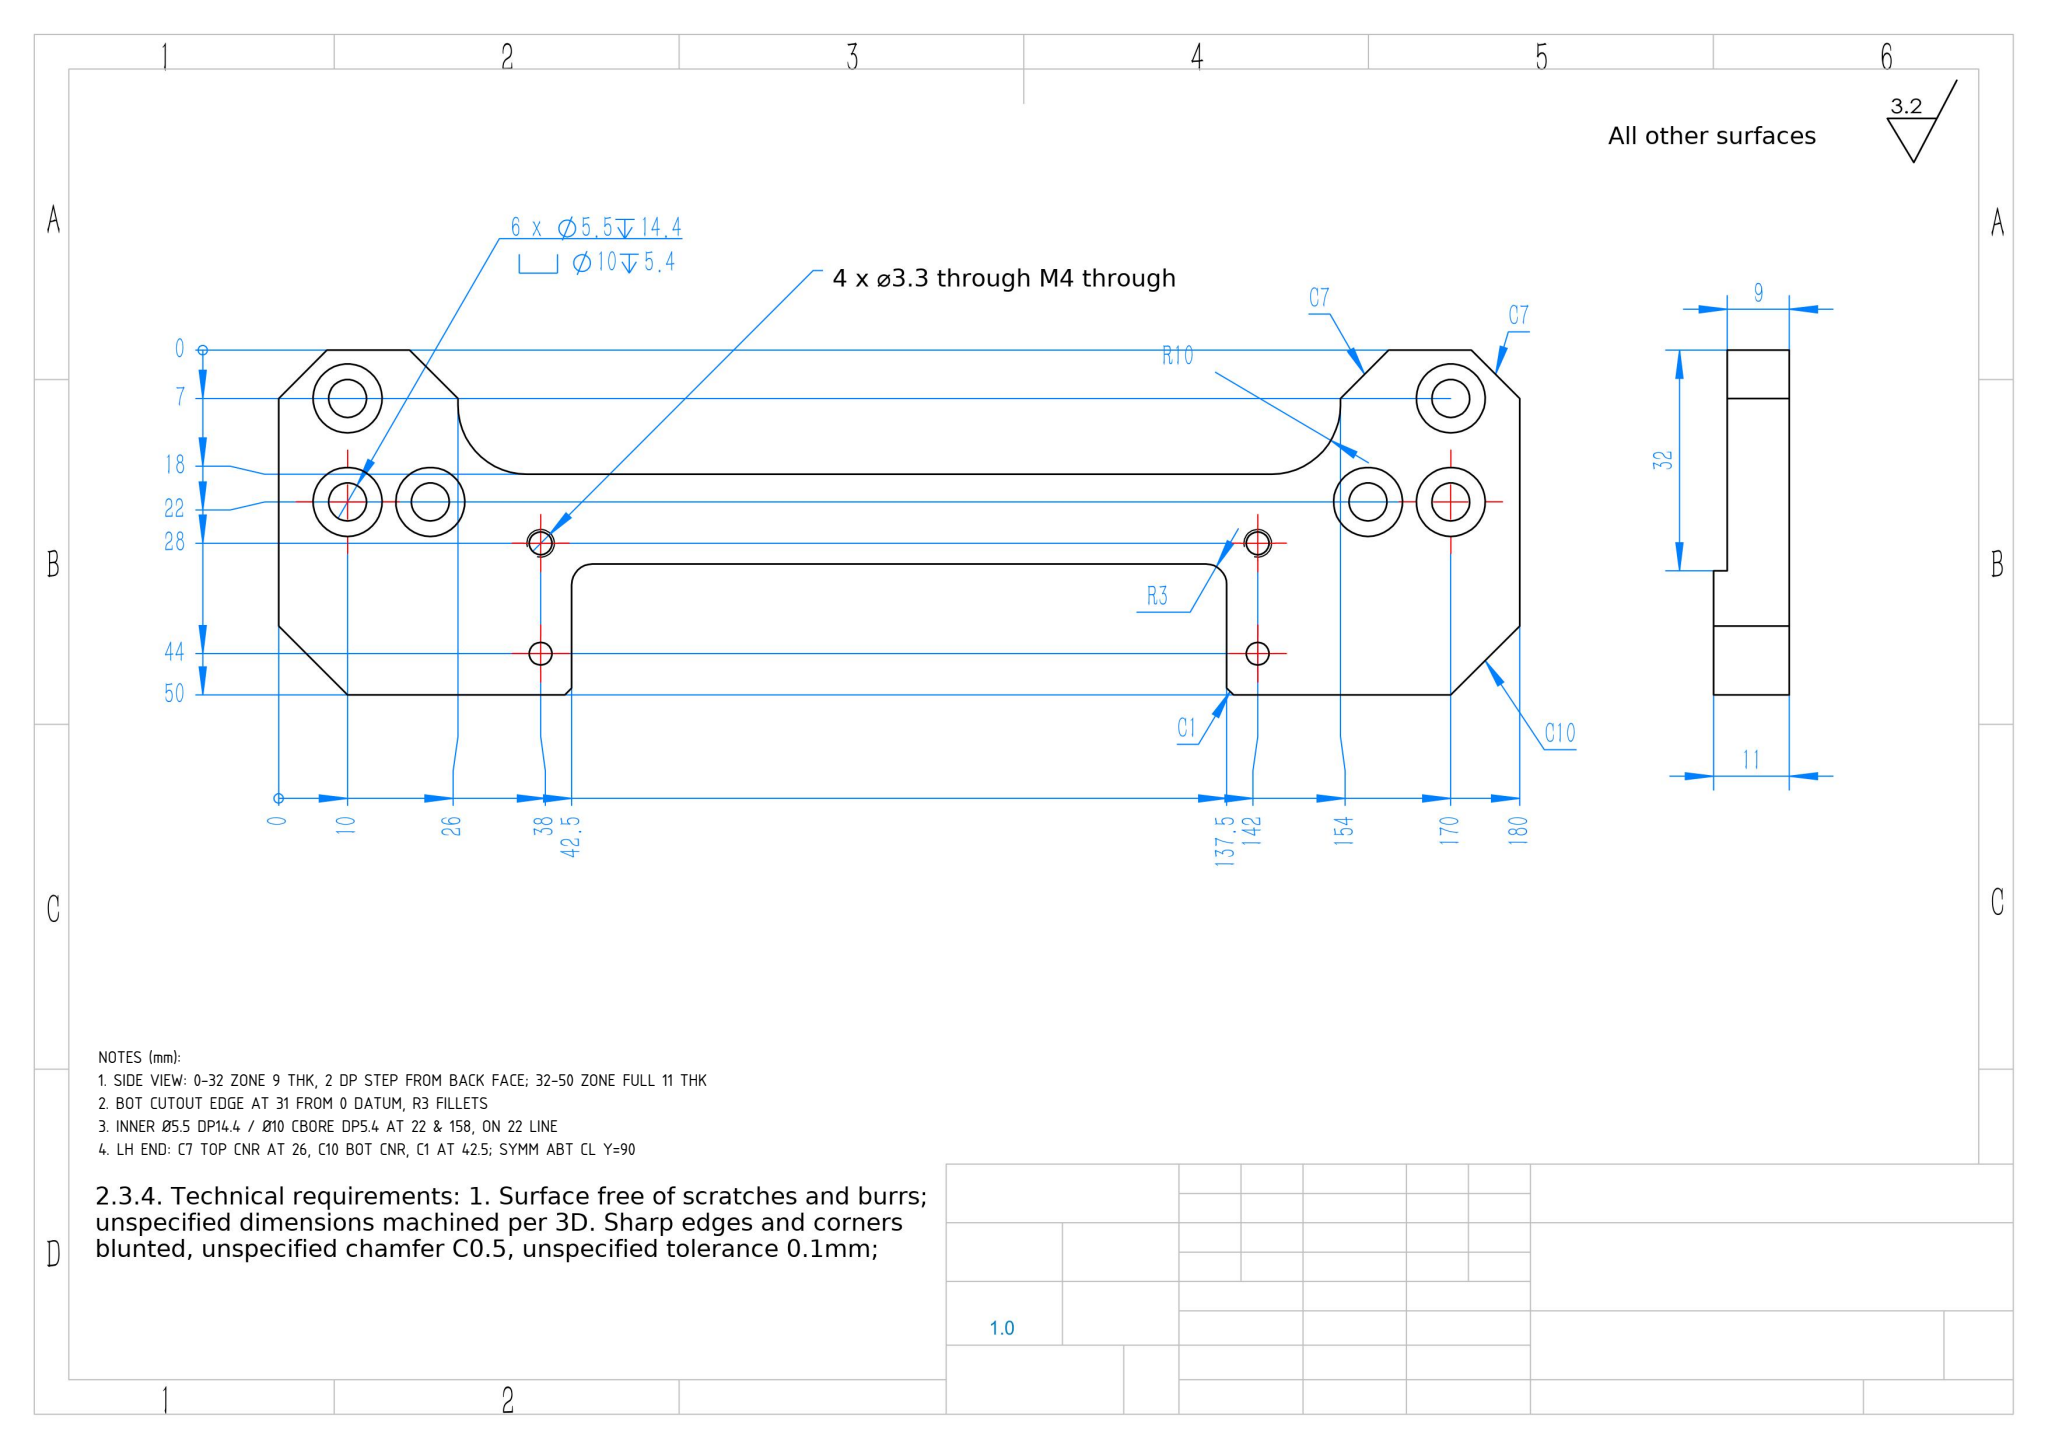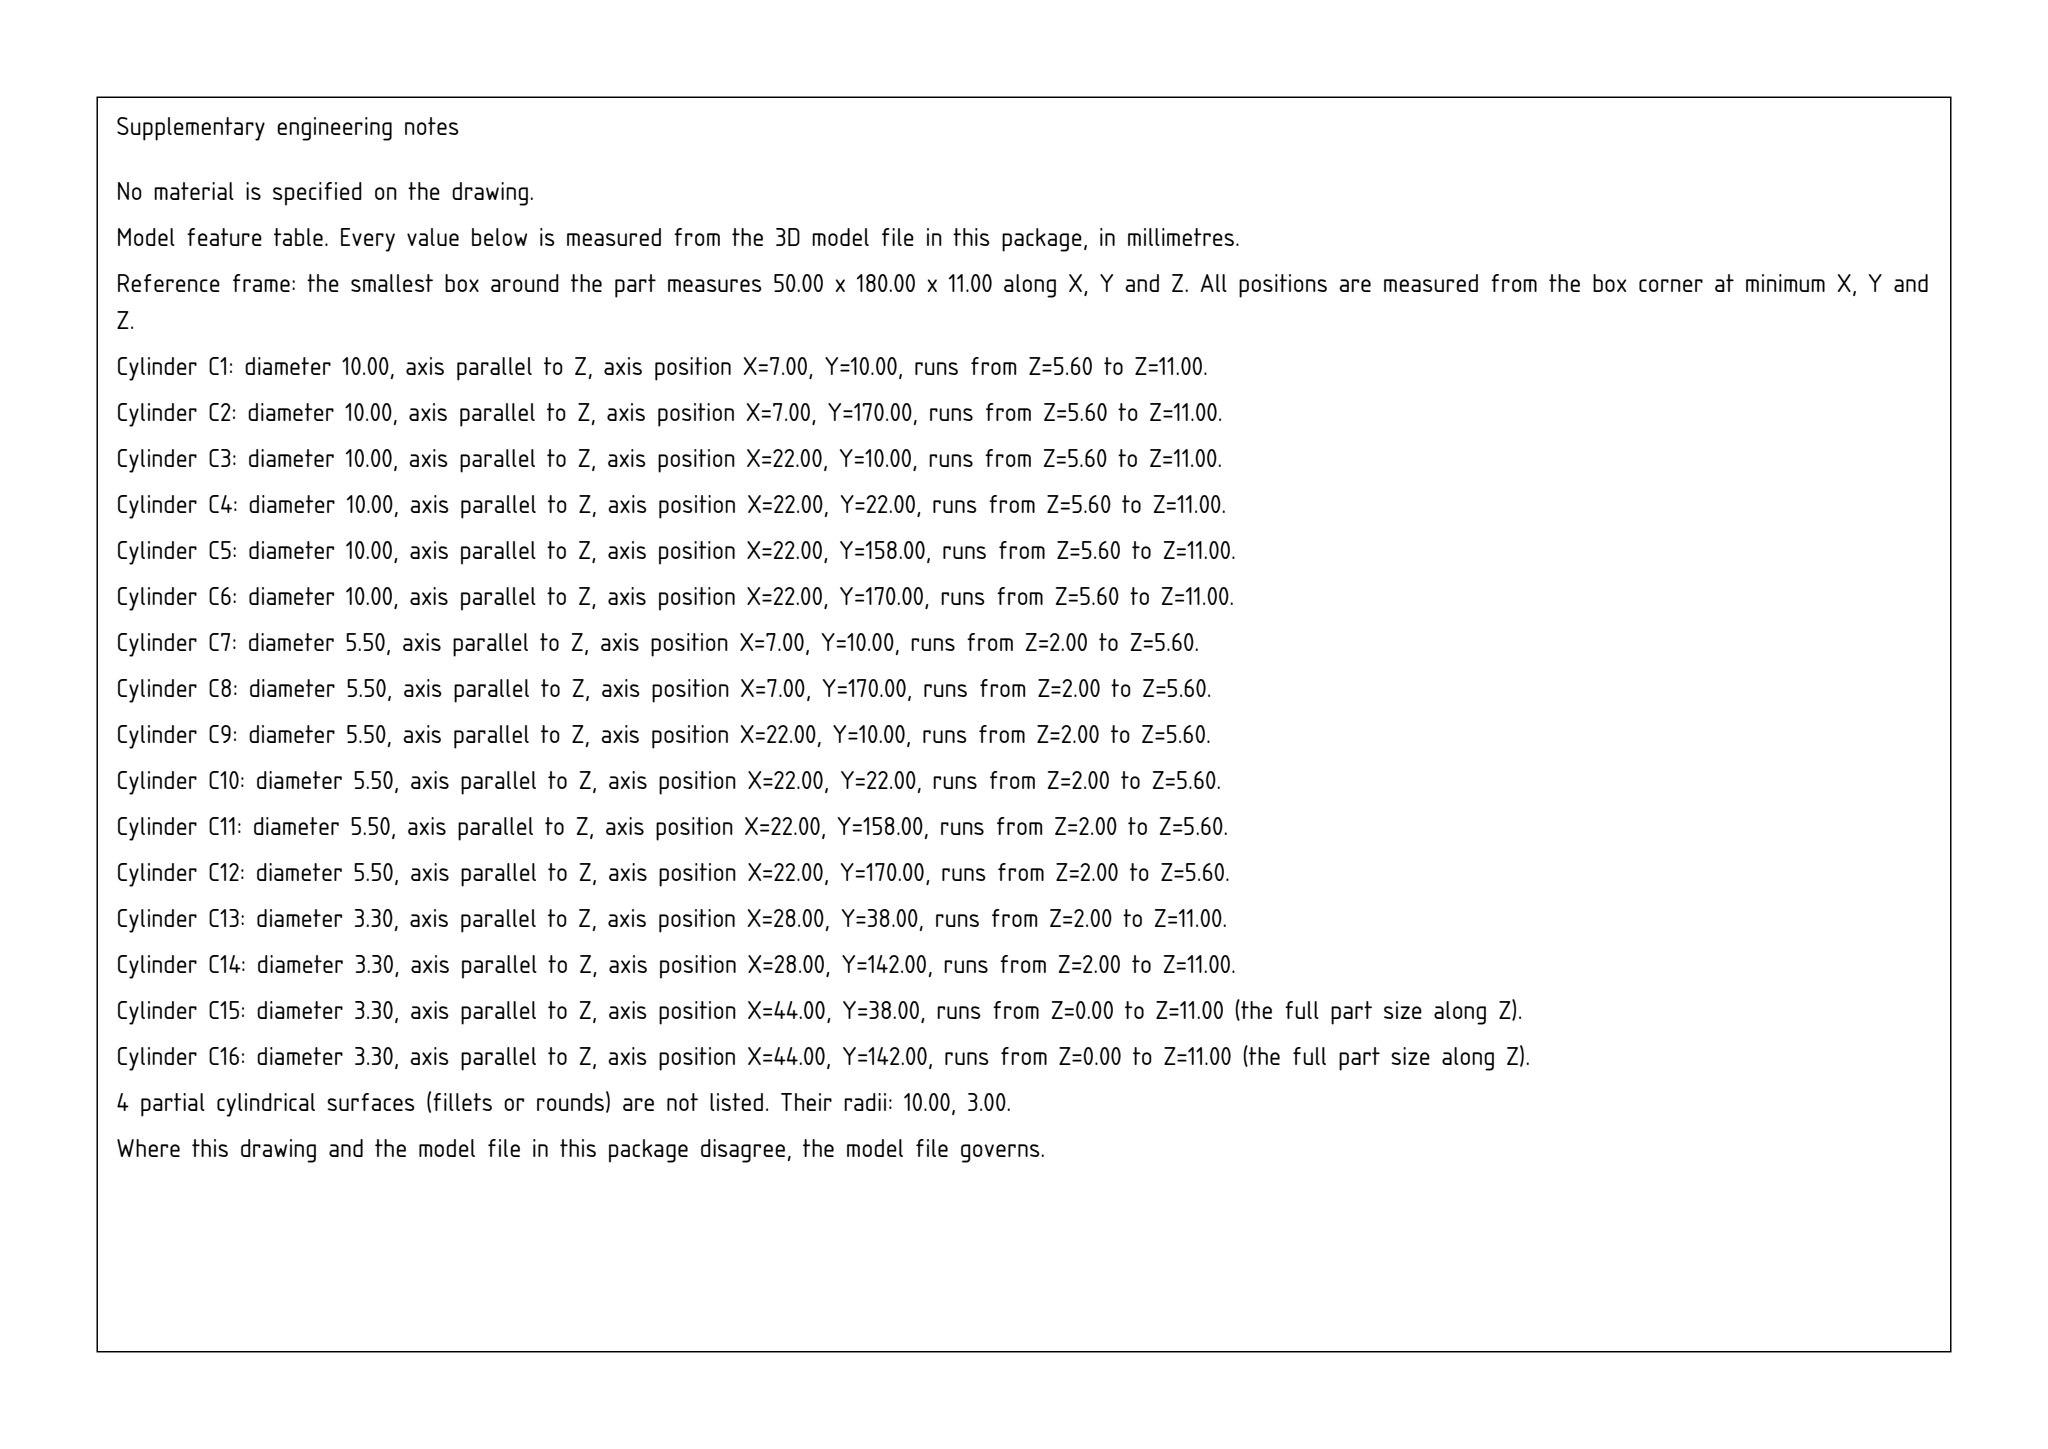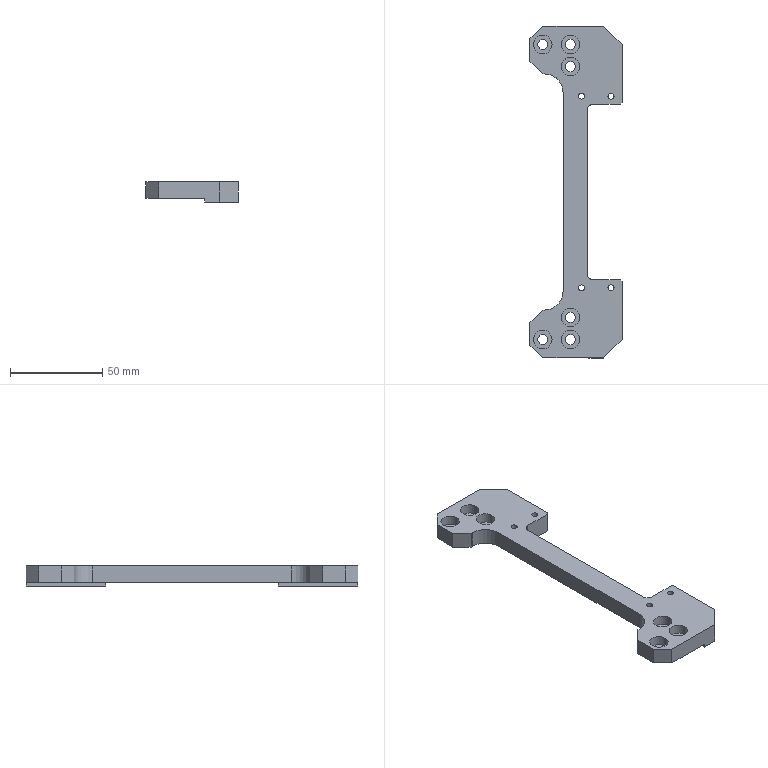Part | SolidWorks | mm | 1 solid | 68 faces | box 50 x 180 x 11 mm | volume 42109 mm3 | cylinder 36 | plane 32 | commonest cylinder face diameters 10 x12 5.5 x12 3.3 x8 20 x2 6 x2
Drawing notes:
SIDE VIEW: 0-32 ZONE 9 THK, 2 DP STEP FROM BACK FACE; 32-50 ZONE FULL 11 THK | from the solid: Z planes 0/2/11; X=32 plane splits zones; Ø3.3 len 9 at X28, len 11 at X44
BOT CUTOUT EDGE AT 31 FROM 0 DATUM, R3 FILLETS | from the solid: axis_plane x=31.0 (cutout face) with datum x=0.0; R3 callout at cutout cnrs
INNER Ø5.5 DP14.4 / Ø10 CBORE DP5.4 AT 22 & 158, ON 22 LINE | from the solid: Ø5.5 & Ø10 z-cylinders at (22,22) and (22,158); bbox Y=180, 158=180-22
LH END: C7 TOP CNR AT 26, C10 BOT CNR, C1 AT 42.5; SYMM ABT CL Y=90 | from the solid: Y planes 26/42.5 mirror 154/137.5 carrying C7 and C1 on RH end; profile symm
build123d program:
from build123d import *

# Parameters (mm, degrees)
SKETCH1_W                                       = 50
SKETCH1_H                                       = 180
BOSS_EXTRUDE1_DEPTH                             = 5.5
SKETCH2_W                                       = 36
SKETCH2_H                                       = 128
CUT_EXTRUDE1_DEPTH                              = 95.053
SKETCH4_W                                       = 32
SKETCH4_H                                       = 2
CUT_EXTRUDE3_DEPTH                              = 182.811
M5_HEX_SOCKET_HEAD_CAP_SCREW_CBORE1_D           = 5.5
M5_HEX_SOCKET_HEAD_CAP_SCREW_CBORE1_DEPTH       = 14.4
M5_HEX_SOCKET_HEAD_CAP_SCREW_CBORE1_CBORE_D     = 10
M5_HEX_SOCKET_HEAD_CAP_SCREW_CBORE1_CBORE_DEPTH = 5.4
M5_HEX_SOCKET_HEAD_CAP_SCREW_CBORE1_TIP         = 1.652
CHAMFER1_SIZE                                   = 7
SKETCH7_W                                       = 38
SKETCH7_H                                       = 95
CUT_EXTRUDE4_DEPTH                              = 95.053
CHAMFER2_SIZE                                   = 1
M4_TAPPED_HOLE1_D                               = 3.3
FILLET1_R                                       = 10
FILLET2_R                                       = 3
CHAMFER3_SIZE                                   = 10


with BuildPart() as part:
    # Sketch1 → Boss-Extrude1 (new, symmetric)
    with BuildSketch(Plane.XY):
        Rectangle(SKETCH1_W, SKETCH1_H)
    extrude(amount=BOSS_EXTRUDE1_DEPTH, both=True)

    # Sketch2 → Cut-Extrude1 (cut, through all)
    with BuildSketch(Plane.XY.offset(5.5)):
        with Locations((-25, 0)):
            Rectangle(SKETCH2_W, SKETCH2_H)
    extrude(amount=-CUT_EXTRUDE1_DEPTH, mode=Mode.SUBTRACT)

    # Sketch4 → Cut-Extrude3 (cut, through all)
    with BuildSketch(Plane.XZ.offset(90)):
        with Locations((-9, -4.5)):
            Rectangle(SKETCH4_W, SKETCH4_H)
    extrude(amount=-CUT_EXTRUDE3_DEPTH, mode=Mode.SUBTRACT)

    # M5 Hex Socket Head Cap Screw CBORE1
    with Locations(Plane.XY.offset(5.5)):
        with Locations((-3, -80), (-3, 80), (-18, -80), (-18, 80), (-3, -68), (-3, 68)):
            CounterBoreHole(M5_HEX_SOCKET_HEAD_CAP_SCREW_CBORE1_D / 2, M5_HEX_SOCKET_HEAD_CAP_SCREW_CBORE1_CBORE_D / 2, M5_HEX_SOCKET_HEAD_CAP_SCREW_CBORE1_CBORE_DEPTH, depth=M5_HEX_SOCKET_HEAD_CAP_SCREW_CBORE1_DEPTH)
            with Locations((0, 0, -(M5_HEX_SOCKET_HEAD_CAP_SCREW_CBORE1_DEPTH + M5_HEX_SOCKET_HEAD_CAP_SCREW_CBORE1_TIP / 2))):  # 118° drill point
                Cone(0, M5_HEX_SOCKET_HEAD_CAP_SCREW_CBORE1_D / 2, M5_HEX_SOCKET_HEAD_CAP_SCREW_CBORE1_TIP, mode=Mode.SUBTRACT)

    # Chamfer1
    chamfer1_edges = [part.edges().sort_by_distance(p)[0] for p in [
        (-25, -64, 1),
        (-25, 64, 1),
        (-25, -90, 1),
        (-25, 90, 1),
    ]]
    chamfer(chamfer1_edges, length=CHAMFER1_SIZE)

    # Sketch7 → Cut-Extrude4 (cut, through all)
    with BuildSketch(Plane.XY.offset(5.5)):
        with Locations((25, 0)):
            Rectangle(SKETCH7_W, SKETCH7_H)
    extrude(amount=-CUT_EXTRUDE4_DEPTH, mode=Mode.SUBTRACT)

    # Chamfer2
    chamfer2_edges = [part.edges().sort_by_distance(p)[0] for p in [
        (25, 47.5, 0),
        (25, -47.5, 0),
    ]]
    chamfer(chamfer2_edges, length=CHAMFER2_SIZE)

    # M4 Tapped Hole1 (through all)
    with Locations(Plane.XY.offset(5.5)):
        with Locations((3, -52), (19, -52), (3, 52), (19, 52)):
            Hole(M4_TAPPED_HOLE1_D / 2)

    # Fillet1
    fillet1_edges = [part.edges().sort_by_distance(p)[0] for p in [
        (-7, 64, 1),
        (-7, -64, 1),
    ]]
    fillet(fillet1_edges, radius=FILLET1_R)

    # Fillet2
    fillet2_edges = [part.edges().sort_by_distance(p)[0] for p in [
        (6, 47.5, 1),
        (6, -47.5, 1),
    ]]
    fillet(fillet2_edges, radius=FILLET2_R)

    # Chamfer3
    chamfer3_edges = [part.edges().sort_by_distance(p)[0] for p in [
        (25, -90, 0),
        (25, 90, 0),
    ]]
    chamfer(chamfer3_edges, length=CHAMFER3_SIZE)


solid = part.part